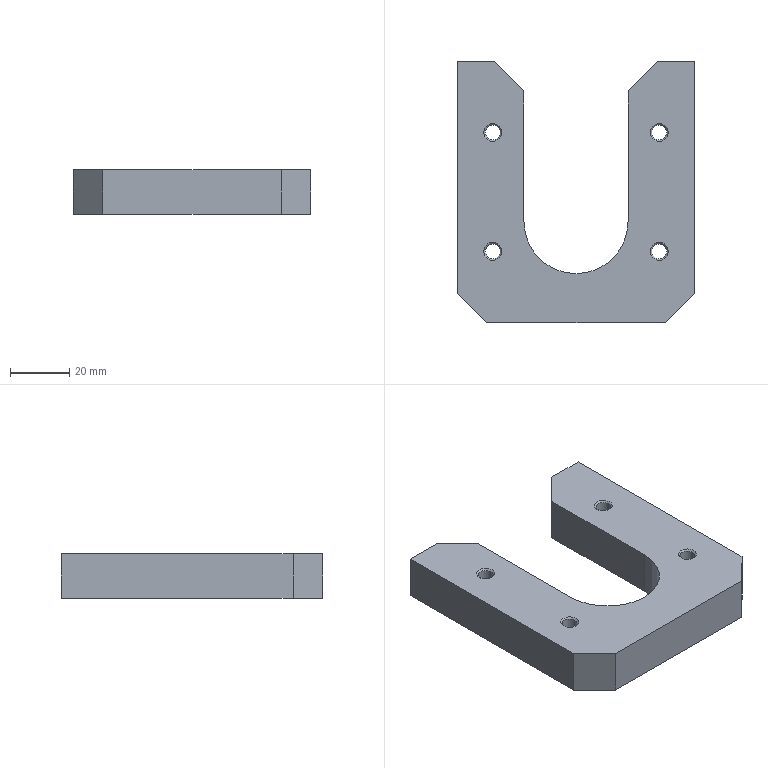Component | SolidWorks | StopBlock-2 | 1 solid | 30 faces | box 80 x 88 x 15 mm | volume 65847 mm3 | plane 13 | cylinder 9 | cone 8 | commonest cylinder face diameters 5 x8 35 x1
build123d program:
from build123d import *

# Parameters (mm, degrees)
SKETCH1_W                = 80
SKETCH1_H                = 88
BOSS_EXTRUDE1_DEPTH      = 15
CUT_EXTRUDE1_DEPTH       = 98.821
F_5_0_5_DIAMETER_HOLE1_D = 5
CHAMFER1_SIZE            = 0.525
CHAMFER2_SIZE            = 10


with BuildPart() as part:
    # Sketch1 → Boss-Extrude1 (new body)
    with BuildSketch(Plane.XY.offset(7.5)):
        with Locations((0, 44)):
            Rectangle(SKETCH1_W, SKETCH1_H)
    extrude(amount=-BOSS_EXTRUDE1_DEPTH)

    # Sketch2 → Cut-Extrude1 (cut, through all)
    with BuildSketch(Plane(origin=(0, 0, -7.5), x_dir=(-1, 0, 0), z_dir=(0, 0, -1))):
        with BuildLine():
            Line((-27.5, 88), (-17.5, 78))
            Line((-17.5, 78), (-17.5, 34))
            ThreePointArc((-17.5, 34), (0, 16.5), (17.5, 34))
            Line((17.5, 34), (17.5, 78))
            Line((17.5, 78), (27.5, 88))
            Line((27.5, 88), (-27.5, 88))
        make_face()
    extrude(amount=-CUT_EXTRUDE1_DEPTH, mode=Mode.SUBTRACT)

    # 5.0 _5_ Diameter Hole1 (through all)
    with Locations(Plane.XY.offset(7.5)):
        with Locations((-28, 24), (28, 24), (28, 64), (-28, 64)):
            Hole(F_5_0_5_DIAMETER_HOLE1_D / 2)

    # Chamfer1
    chamfer1_edges = [part.edges().sort_by_distance(p)[0] for p in [
        (-25.5, 64, 7.5),
        (30.5, 64, 7.5),
        (30.5, 24, 7.5),
        (-25.5, 24, 7.5),
    ]]
    chamfer(chamfer1_edges, length=CHAMFER1_SIZE)

    # Chamfer2
    chamfer2_edges = [part.edges().sort_by_distance(p)[0] for p in [
        (40, 0, 0),
        (-40, 0, 0),
    ]]
    chamfer(chamfer2_edges, length=CHAMFER2_SIZE)


solid = part.part

# Placed as in the assembly
solid = solid.moved(Location((-345, -263, -255), (0, 0, 0)))
STEP:
#1=CARTESIAN_POINT('',(-12.579,-7.835,-9.765));
#2=VERTEX_POINT('',#1);
#3=CARTESIAN_POINT('',(-12.382,-7.835,-9.765));
#4=VERTEX_POINT('',#3);
#5=CARTESIAN_POINT('',(-12.48,-7.835,-9.765));
#6=DIRECTION('',(0.,0.,1.));
#7=DIRECTION('',(1.,0.,0.));
#8=AXIS2_PLACEMENT_3D('',#5,#6,#7);
#9=CIRCLE('',#8,0.09843);
#10=EDGE_CURVE('',#2,#4,#9,.T.);
#11=ORIENTED_EDGE('',*,*,#10,.F.);
#12=CARTESIAN_POINT('',(-12.599,-7.835,-9.744));
#13=VERTEX_POINT('',#12);
#14=CARTESIAN_POINT('',(-12.579,-7.835,-9.765));
#15=DIRECTION('',(-0.7071,0.,0.7071));
#16=VECTOR('',#15,39.37);
#17=LINE('',#14,#16);
#18=EDGE_CURVE('',#2,#13,#17,.T.);
#19=ORIENTED_EDGE('',*,*,#18,.T.);
#20=CARTESIAN_POINT('',(-12.361,-7.835,-9.744));
#21=VERTEX_POINT('',#20);
#22=CARTESIAN_POINT('',(-12.48,-7.835,-9.744));
#23=DIRECTION('',(0.,0.,-1.));
#24=DIRECTION('',(1.,0.,0.));
#25=AXIS2_PLACEMENT_3D('',#22,#23,#24);
#26=CIRCLE('',#25,0.1191);
#27=EDGE_CURVE('',#21,#13,#26,.T.);
#28=ORIENTED_EDGE('',*,*,#27,.F.);
#29=CARTESIAN_POINT('',(-12.382,-7.835,-9.765));
#30=DIRECTION('',(0.7071,0.,0.7071));
#31=VECTOR('',#30,39.37);
#32=LINE('',#29,#31);
#33=EDGE_CURVE('',#4,#21,#32,.T.);
#34=ORIENTED_EDGE('',*,*,#33,.F.);
#35=EDGE_LOOP('',(#11,#19,#28,#34));
#36=FACE_OUTER_BOUND('',#35,.T.);
#37=CARTESIAN_POINT('',(-12.48,-7.835,-9.765));
#38=DIRECTION('',(0.,0.,1.));
#39=DIRECTION('',(1.,0.,0.));
#40=AXIS2_PLACEMENT_3D('',#37,#38,#39);
#41=CONICAL_SURFACE('',#40,0.09843,0.7854);
#42=ADVANCED_FACE('',(#36),#41,.F.);
#43=CARTESIAN_POINT('',(-14.783,-9.409,-9.765));
#44=VERTEX_POINT('',#43);
#45=CARTESIAN_POINT('',(-14.587,-9.409,-9.765));
#46=VERTEX_POINT('',#45);
#47=CARTESIAN_POINT('',(-14.685,-9.409,-9.765));
#48=DIRECTION('',(0.,0.,1.));
#49=DIRECTION('',(1.,0.,0.));
#50=AXIS2_PLACEMENT_3D('',#47,#48,#49);
#51=CIRCLE('',#50,0.09843);
#52=EDGE_CURVE('',#44,#46,#51,.T.);
#53=ORIENTED_EDGE('',*,*,#52,.F.);
#54=CARTESIAN_POINT('',(-14.804,-9.409,-9.744));
#55=VERTEX_POINT('',#54);
#56=CARTESIAN_POINT('',(-14.783,-9.409,-9.765));
#57=DIRECTION('',(-0.7071,0.,0.7071));
#58=VECTOR('',#57,39.37);
#59=LINE('',#56,#58);
#60=EDGE_CURVE('',#44,#55,#59,.T.);
#61=ORIENTED_EDGE('',*,*,#60,.T.);
#62=CARTESIAN_POINT('',(-14.566,-9.409,-9.744));
#63=VERTEX_POINT('',#62);
#64=CARTESIAN_POINT('',(-14.685,-9.409,-9.744));
#65=DIRECTION('',(0.,0.,-1.));
#66=DIRECTION('',(1.,0.,0.));
#67=AXIS2_PLACEMENT_3D('',#64,#65,#66);
#68=CIRCLE('',#67,0.1191);
#69=EDGE_CURVE('',#63,#55,#68,.T.);
#70=ORIENTED_EDGE('',*,*,#69,.F.);
#71=CARTESIAN_POINT('',(-14.587,-9.409,-9.765));
#72=DIRECTION('',(0.7071,0.,0.7071));
#73=VECTOR('',#72,39.37);
#74=LINE('',#71,#73);
#75=EDGE_CURVE('',#46,#63,#74,.T.);
#76=ORIENTED_EDGE('',*,*,#75,.F.);
#77=EDGE_LOOP('',(#53,#61,#70,#76));
#78=FACE_OUTER_BOUND('',#77,.T.);
#79=CARTESIAN_POINT('',(-14.685,-9.409,-9.765));
#80=DIRECTION('',(0.,0.,1.));
#81=DIRECTION('',(1.,0.,0.));
#82=AXIS2_PLACEMENT_3D('',#79,#80,#81);
#83=CONICAL_SURFACE('',#82,0.09843,0.7854);
#84=ADVANCED_FACE('',(#78),#83,.F.);
#85=CARTESIAN_POINT('',(-12.579,-9.409,-9.765));
#86=VERTEX_POINT('',#85);
#87=CARTESIAN_POINT('',(-12.382,-9.409,-9.765));
#88=VERTEX_POINT('',#87);
#89=CARTESIAN_POINT('',(-12.48,-9.409,-9.765));
#90=DIRECTION('',(0.,0.,1.));
#91=DIRECTION('',(1.,0.,0.));
#92=AXIS2_PLACEMENT_3D('',#89,#90,#91);
#93=CIRCLE('',#92,0.09843);
#94=EDGE_CURVE('',#86,#88,#93,.T.);
#95=ORIENTED_EDGE('',*,*,#94,.F.);
#96=CARTESIAN_POINT('',(-12.599,-9.409,-9.744));
#97=VERTEX_POINT('',#96);
#98=CARTESIAN_POINT('',(-12.579,-9.409,-9.765));
#99=DIRECTION('',(-0.7071,0.,0.7071));
#100=VECTOR('',#99,39.37);
#101=LINE('',#98,#100);
#102=EDGE_CURVE('',#86,#97,#101,.T.);
#103=ORIENTED_EDGE('',*,*,#102,.T.);
#104=CARTESIAN_POINT('',(-12.361,-9.409,-9.744));
#105=VERTEX_POINT('',#104);
#106=CARTESIAN_POINT('',(-12.48,-9.409,-9.744));
#107=DIRECTION('',(0.,0.,-1.));
#108=DIRECTION('',(1.,0.,0.));
#109=AXIS2_PLACEMENT_3D('',#106,#107,#108);
#110=CIRCLE('',#109,0.1191);
#111=EDGE_CURVE('',#105,#97,#110,.T.);
#112=ORIENTED_EDGE('',*,*,#111,.F.);
#113=CARTESIAN_POINT('',(-12.382,-9.409,-9.765));
#114=DIRECTION('',(0.7071,0.,0.7071));
#115=VECTOR('',#114,39.37);
#116=LINE('',#113,#115);
#117=EDGE_CURVE('',#88,#105,#116,.T.);
#118=ORIENTED_EDGE('',*,*,#117,.F.);
#119=EDGE_LOOP('',(#95,#103,#112,#118));
#120=FACE_OUTER_BOUND('',#119,.T.);
#121=CARTESIAN_POINT('',(-12.48,-9.409,-9.765));
#122=DIRECTION('',(0.,0.,1.));
#123=DIRECTION('',(1.,0.,0.));
#124=AXIS2_PLACEMENT_3D('',#121,#122,#123);
#125=CONICAL_SURFACE('',#124,0.09843,0.7854);
#126=ADVANCED_FACE('',(#120),#125,.F.);
#127=CARTESIAN_POINT('',(-14.783,-7.835,-9.765));
#128=VERTEX_POINT('',#127);
#129=CARTESIAN_POINT('',(-14.587,-7.835,-9.765));
#130=VERTEX_POINT('',#129);
#131=CARTESIAN_POINT('',(-14.685,-7.835,-9.765));
#132=DIRECTION('',(0.,0.,1.));
#133=DIRECTION('',(1.,0.,0.));
#134=AXIS2_PLACEMENT_3D('',#131,#132,#133);
#135=CIRCLE('',#134,0.09843);
#136=EDGE_CURVE('',#128,#130,#135,.T.);
#137=ORIENTED_EDGE('',*,*,#136,.F.);
#138=CARTESIAN_POINT('',(-14.804,-7.835,-9.744));
#139=VERTEX_POINT('',#138);
#140=CARTESIAN_POINT('',(-14.783,-7.835,-9.765));
#141=DIRECTION('',(-0.7071,0.,0.7071));
#142=VECTOR('',#141,39.37);
#143=LINE('',#140,#142);
#144=EDGE_CURVE('',#128,#139,#143,.T.);
#145=ORIENTED_EDGE('',*,*,#144,.T.);
#146=CARTESIAN_POINT('',(-14.566,-7.835,-9.744));
#147=VERTEX_POINT('',#146);
#148=CARTESIAN_POINT('',(-14.685,-7.835,-9.744));
#149=DIRECTION('',(0.,0.,-1.));
#150=DIRECTION('',(1.,0.,0.));
#151=AXIS2_PLACEMENT_3D('',#148,#149,#150);
#152=CIRCLE('',#151,0.1191);
#153=EDGE_CURVE('',#147,#139,#152,.T.);
#154=ORIENTED_EDGE('',*,*,#153,.F.);
#155=CARTESIAN_POINT('',(-14.587,-7.835,-9.765));
#156=DIRECTION('',(0.7071,0.,0.7071));
#157=VECTOR('',#156,39.37);
#158=LINE('',#155,#157);
#159=EDGE_CURVE('',#130,#147,#158,.T.);
#160=ORIENTED_EDGE('',*,*,#159,.F.);
#161=EDGE_LOOP('',(#137,#145,#154,#160));
#162=FACE_OUTER_BOUND('',#161,.T.);
#163=CARTESIAN_POINT('',(-14.685,-7.835,-9.765));
#164=DIRECTION('',(0.,0.,1.));
#165=DIRECTION('',(1.,0.,0.));
#166=AXIS2_PLACEMENT_3D('',#163,#164,#165);
#167=CONICAL_SURFACE('',#166,0.09843,0.7854);
#168=ADVANCED_FACE('',(#162),#167,.F.);
#169=CARTESIAN_POINT('',(-14.783,-9.409,-10.335));
#170=VERTEX_POINT('',#169);
#171=CARTESIAN_POINT('',(-14.587,-9.409,-10.335));
#172=VERTEX_POINT('',#171);
#173=CARTESIAN_POINT('',(-14.685,-9.409,-10.335));
#174=DIRECTION('',(0.,0.,1.));
#175=DIRECTION('',(1.,0.,0.));
#176=AXIS2_PLACEMENT_3D('',#173,#174,#175);
#177=CIRCLE('',#176,0.09843);
#178=EDGE_CURVE('',#170,#172,#177,.T.);
#179=ORIENTED_EDGE('',*,*,#178,.F.);
#180=CARTESIAN_POINT('',(-14.783,-9.409,-9.744));
#181=DIRECTION('',(0.,0.,1.));
#182=VECTOR('',#181,39.37);
#183=LINE('',#180,#182);
#184=EDGE_CURVE('',#170,#44,#183,.T.);
#185=ORIENTED_EDGE('',*,*,#184,.T.);
#186=ORIENTED_EDGE('',*,*,#52,.T.);
#187=CARTESIAN_POINT('',(-14.587,-9.409,-9.744));
#188=DIRECTION('',(0.,0.,1.));
#189=VECTOR('',#188,39.37);
#190=LINE('',#187,#189);
#191=EDGE_CURVE('',#172,#46,#190,.T.);
#192=ORIENTED_EDGE('',*,*,#191,.F.);
#193=EDGE_LOOP('',(#179,#185,#186,#192));
#194=FACE_OUTER_BOUND('',#193,.T.);
#195=CARTESIAN_POINT('',(-14.685,-9.409,-9.744));
#196=DIRECTION('',(0.,0.,1.));
#197=DIRECTION('',(1.,0.,0.));
#198=AXIS2_PLACEMENT_3D('',#195,#196,#197);
#199=CYLINDRICAL_SURFACE('',#198,0.09843);
#200=ADVANCED_FACE('',(#194),#199,.F.);
#201=CARTESIAN_POINT('',(-12.579,-9.409,-10.335));
#202=VERTEX_POINT('',#201);
#203=CARTESIAN_POINT('',(-12.382,-9.409,-10.335));
#204=VERTEX_POINT('',#203);
#205=CARTESIAN_POINT('',(-12.48,-9.409,-10.335));
#206=DIRECTION('',(0.,0.,1.));
#207=DIRECTION('',(1.,0.,0.));
#208=AXIS2_PLACEMENT_3D('',#205,#206,#207);
#209=CIRCLE('',#208,0.09843);
#210=EDGE_CURVE('',#202,#204,#209,.T.);
#211=ORIENTED_EDGE('',*,*,#210,.F.);
#212=CARTESIAN_POINT('',(-12.579,-9.409,-9.744));
#213=DIRECTION('',(0.,0.,1.));
#214=VECTOR('',#213,39.37);
#215=LINE('',#212,#214);
#216=EDGE_CURVE('',#202,#86,#215,.T.);
#217=ORIENTED_EDGE('',*,*,#216,.T.);
#218=ORIENTED_EDGE('',*,*,#94,.T.);
#219=CARTESIAN_POINT('',(-12.382,-9.409,-9.744));
#220=DIRECTION('',(0.,0.,1.));
#221=VECTOR('',#220,39.37);
#222=LINE('',#219,#221);
#223=EDGE_CURVE('',#204,#88,#222,.T.);
#224=ORIENTED_EDGE('',*,*,#223,.F.);
#225=EDGE_LOOP('',(#211,#217,#218,#224));
#226=FACE_OUTER_BOUND('',#225,.T.);
#227=CARTESIAN_POINT('',(-12.48,-9.409,-9.744));
#228=DIRECTION('',(0.,0.,1.));
#229=DIRECTION('',(1.,0.,0.));
#230=AXIS2_PLACEMENT_3D('',#227,#228,#229);
#231=CYLINDRICAL_SURFACE('',#230,0.09843);
#232=ADVANCED_FACE('',(#226),#231,.F.);
#233=CARTESIAN_POINT('',(-12.579,-7.835,-10.335));
#234=VERTEX_POINT('',#233);
#235=CARTESIAN_POINT('',(-12.382,-7.835,-10.335));
#236=VERTEX_POINT('',#235);
#237=CARTESIAN_POINT('',(-12.48,-7.835,-10.335));
#238=DIRECTION('',(0.,0.,1.));
#239=DIRECTION('',(1.,0.,0.));
#240=AXIS2_PLACEMENT_3D('',#237,#238,#239);
#241=CIRCLE('',#240,0.09843);
#242=EDGE_CURVE('',#234,#236,#241,.T.);
#243=ORIENTED_EDGE('',*,*,#242,.F.);
#244=CARTESIAN_POINT('',(-12.579,-7.835,-9.744));
#245=DIRECTION('',(0.,0.,1.));
#246=VECTOR('',#245,39.37);
#247=LINE('',#244,#246);
#248=EDGE_CURVE('',#234,#2,#247,.T.);
#249=ORIENTED_EDGE('',*,*,#248,.T.);
#250=ORIENTED_EDGE('',*,*,#10,.T.);
#251=CARTESIAN_POINT('',(-12.382,-7.835,-9.744));
#252=DIRECTION('',(0.,0.,1.));
#253=VECTOR('',#252,39.37);
#254=LINE('',#251,#253);
#255=EDGE_CURVE('',#236,#4,#254,.T.);
#256=ORIENTED_EDGE('',*,*,#255,.F.);
#257=EDGE_LOOP('',(#243,#249,#250,#256));
#258=FACE_OUTER_BOUND('',#257,.T.);
#259=CARTESIAN_POINT('',(-12.48,-7.835,-9.744));
#260=DIRECTION('',(0.,0.,1.));
#261=DIRECTION('',(1.,0.,0.));
#262=AXIS2_PLACEMENT_3D('',#259,#260,#261);
#263=CYLINDRICAL_SURFACE('',#262,0.09843);
#264=ADVANCED_FACE('',(#258),#263,.F.);
#265=CARTESIAN_POINT('',(-14.783,-7.835,-10.335));
#266=VERTEX_POINT('',#265);
#267=CARTESIAN_POINT('',(-14.587,-7.835,-10.335));
#268=VERTEX_POINT('',#267);
#269=CARTESIAN_POINT('',(-14.685,-7.835,-10.335));
#270=DIRECTION('',(0.,0.,1.));
#271=DIRECTION('',(1.,0.,0.));
#272=AXIS2_PLACEMENT_3D('',#269,#270,#271);
#273=CIRCLE('',#272,0.09843);
#274=EDGE_CURVE('',#266,#268,#273,.T.);
#275=ORIENTED_EDGE('',*,*,#274,.F.);
#276=CARTESIAN_POINT('',(-14.783,-7.835,-9.744));
#277=DIRECTION('',(0.,0.,1.));
#278=VECTOR('',#277,39.37);
#279=LINE('',#276,#278);
#280=EDGE_CURVE('',#266,#128,#279,.T.);
#281=ORIENTED_EDGE('',*,*,#280,.T.);
#282=ORIENTED_EDGE('',*,*,#136,.T.);
#283=CARTESIAN_POINT('',(-14.587,-7.835,-9.744));
#284=DIRECTION('',(0.,0.,1.));
#285=VECTOR('',#284,39.37);
#286=LINE('',#283,#285);
#287=EDGE_CURVE('',#268,#130,#286,.T.);
#288=ORIENTED_EDGE('',*,*,#287,.F.);
#289=EDGE_LOOP('',(#275,#281,#282,#288));
#290=FACE_OUTER_BOUND('',#289,.T.);
#291=CARTESIAN_POINT('',(-14.685,-7.835,-9.744));
#292=DIRECTION('',(0.,0.,1.));
#293=DIRECTION('',(1.,0.,0.));
#294=AXIS2_PLACEMENT_3D('',#291,#292,#293);
#295=CYLINDRICAL_SURFACE('',#294,0.09843);
#296=ADVANCED_FACE('',(#290),#295,.F.);
#297=CARTESIAN_POINT('',(-14.665,-6.89,-9.744));
#298=VERTEX_POINT('',#297);
#299=CARTESIAN_POINT('',(-14.665,-6.89,-10.335));
#300=VERTEX_POINT('',#299);
#301=CARTESIAN_POINT('',(-14.665,-6.89,-9.744));
#302=DIRECTION('',(0.,0.,-1.));
#303=VECTOR('',#302,39.37);
#304=LINE('',#301,#303);
#305=EDGE_CURVE('',#298,#300,#304,.T.);
#306=ORIENTED_EDGE('',*,*,#305,.T.);
#307=CARTESIAN_POINT('',(-15.157,-6.89,-10.335));
#308=VERTEX_POINT('',#307);
#309=CARTESIAN_POINT('',(-12.008,-6.89,-10.335));
#310=DIRECTION('',(-1.,0.,0.));
#311=VECTOR('',#310,39.37);
#312=LINE('',#309,#311);
#313=EDGE_CURVE('',#300,#308,#312,.T.);
#314=ORIENTED_EDGE('',*,*,#313,.T.);
#315=CARTESIAN_POINT('',(-15.157,-6.89,-9.744));
#316=VERTEX_POINT('',#315);
#317=CARTESIAN_POINT('',(-15.157,-6.89,-10.335));
#318=DIRECTION('',(0.,0.,1.));
#319=VECTOR('',#318,39.37);
#320=LINE('',#317,#319);
#321=EDGE_CURVE('',#308,#316,#320,.T.);
#322=ORIENTED_EDGE('',*,*,#321,.T.);
#323=CARTESIAN_POINT('',(-12.008,-6.89,-9.744));
#324=DIRECTION('',(-1.,0.,0.));
#325=VECTOR('',#324,39.37);
#326=LINE('',#323,#325);
#327=EDGE_CURVE('',#298,#316,#326,.T.);
#328=ORIENTED_EDGE('',*,*,#327,.F.);
#329=EDGE_LOOP('',(#306,#314,#322,#328));
#330=FACE_OUTER_BOUND('',#329,.T.);
#331=CARTESIAN_POINT('',(-12.008,-6.89,-10.335));
#332=DIRECTION('',(0.,1.,0.));
#333=DIRECTION('',(0.,0.,1.));
#334=AXIS2_PLACEMENT_3D('',#331,#332,#333);
#335=PLANE('',#334);
#336=ADVANCED_FACE('',(#330),#335,.T.);
#337=CARTESIAN_POINT('',(-12.008,-9.961,-9.744));
#338=VERTEX_POINT('',#337);
#339=CARTESIAN_POINT('',(-12.008,-6.89,-9.744));
#340=VERTEX_POINT('',#339);
#341=CARTESIAN_POINT('',(-12.008,-10.354,-9.744));
#342=DIRECTION('',(-0.,1.,0.));
#343=VECTOR('',#342,39.37);
#344=LINE('',#341,#343);
#345=EDGE_CURVE('',#338,#340,#344,.T.);
#346=ORIENTED_EDGE('',*,*,#345,.F.);
#347=CARTESIAN_POINT('',(-12.008,-9.961,-10.335));
#348=VERTEX_POINT('',#347);
#349=CARTESIAN_POINT('',(-12.008,-9.961,-10.335));
#350=DIRECTION('',(0.,0.,-1.));
#351=VECTOR('',#350,39.37);
#352=LINE('',#349,#351);
#353=EDGE_CURVE('',#338,#348,#352,.T.);
#354=ORIENTED_EDGE('',*,*,#353,.T.);
#355=CARTESIAN_POINT('',(-12.008,-6.89,-10.335));
#356=VERTEX_POINT('',#355);
#357=CARTESIAN_POINT('',(-12.008,-10.354,-10.335));
#358=DIRECTION('',(-0.,1.,0.));
#359=VECTOR('',#358,39.37);
#360=LINE('',#357,#359);
#361=EDGE_CURVE('',#348,#356,#360,.T.);
#362=ORIENTED_EDGE('',*,*,#361,.T.);
#363=CARTESIAN_POINT('',(-12.008,-6.89,-10.335));
#364=DIRECTION('',(0.,0.,1.));
#365=VECTOR('',#364,39.37);
#366=LINE('',#363,#365);
#367=EDGE_CURVE('',#356,#340,#366,.T.);
#368=ORIENTED_EDGE('',*,*,#367,.T.);
#369=EDGE_LOOP('',(#346,#354,#362,#368));
#370=FACE_OUTER_BOUND('',#369,.T.);
#371=CARTESIAN_POINT('',(-12.008,-10.354,-10.335));
#372=DIRECTION('',(1.,0.,0.));
#373=DIRECTION('',(-0.,1.,0.));
#374=AXIS2_PLACEMENT_3D('',#371,#372,#373);
#375=PLANE('',#374);
#376=ADVANCED_FACE('',(#370),#375,.T.);
#377=CARTESIAN_POINT('',(-14.764,-10.354,-10.335));
#378=VERTEX_POINT('',#377);
#379=CARTESIAN_POINT('',(-12.402,-10.354,-10.335));
#380=VERTEX_POINT('',#379);
#381=CARTESIAN_POINT('',(-15.157,-10.354,-10.335));
#382=DIRECTION('',(1.,0.,0.));
#383=VECTOR('',#382,39.37);
#384=LINE('',#381,#383);
#385=EDGE_CURVE('',#378,#380,#384,.T.);
#386=ORIENTED_EDGE('',*,*,#385,.T.);
#387=CARTESIAN_POINT('',(-12.402,-10.354,-9.744));
#388=VERTEX_POINT('',#387);
#389=CARTESIAN_POINT('',(-12.402,-10.354,-10.335));
#390=DIRECTION('',(0.,0.,1.));
#391=VECTOR('',#390,39.37);
#392=LINE('',#389,#391);
#393=EDGE_CURVE('',#380,#388,#392,.T.);
#394=ORIENTED_EDGE('',*,*,#393,.T.);
#395=CARTESIAN_POINT('',(-14.764,-10.354,-9.744));
#396=VERTEX_POINT('',#395);
#397=CARTESIAN_POINT('',(-15.157,-10.354,-9.744));
#398=DIRECTION('',(1.,0.,0.));
#399=VECTOR('',#398,39.37);
#400=LINE('',#397,#399);
#401=EDGE_CURVE('',#396,#388,#400,.T.);
#402=ORIENTED_EDGE('',*,*,#401,.F.);
#403=CARTESIAN_POINT('',(-14.764,-10.354,-10.335));
#404=DIRECTION('',(0.,0.,-1.));
#405=VECTOR('',#404,39.37);
#406=LINE('',#403,#405);
#407=EDGE_CURVE('',#396,#378,#406,.T.);
#408=ORIENTED_EDGE('',*,*,#407,.T.);
#409=EDGE_LOOP('',(#386,#394,#402,#408));
#410=FACE_OUTER_BOUND('',#409,.T.);
#411=CARTESIAN_POINT('',(-15.157,-10.354,-10.335));
#412=DIRECTION('',(0.,-1.,0.));
#413=DIRECTION('',(0.,0.,-1.));
#414=AXIS2_PLACEMENT_3D('',#411,#412,#413);
#415=PLANE('',#414);
#416=ADVANCED_FACE('',(#410),#415,.T.);
#417=CARTESIAN_POINT('',(-15.157,-9.961,-10.335));
#418=VERTEX_POINT('',#417);
#419=CARTESIAN_POINT('',(-15.157,-6.89,-10.335));
#420=DIRECTION('',(0.,-1.,0.));
#421=VECTOR('',#420,39.37);
#422=LINE('',#419,#421);
#423=EDGE_CURVE('',#308,#418,#422,.T.);
#424=ORIENTED_EDGE('',*,*,#423,.T.);
#425=CARTESIAN_POINT('',(-15.157,-9.961,-9.744));
#426=VERTEX_POINT('',#425);
#427=CARTESIAN_POINT('',(-15.157,-9.961,-10.335));
#428=DIRECTION('',(0.,0.,1.));
#429=VECTOR('',#428,39.37);
#430=LINE('',#427,#429);
#431=EDGE_CURVE('',#418,#426,#430,.T.);
#432=ORIENTED_EDGE('',*,*,#431,.T.);
#433=CARTESIAN_POINT('',(-15.157,-6.89,-9.744));
#434=DIRECTION('',(0.,-1.,0.));
#435=VECTOR('',#434,39.37);
#436=LINE('',#433,#435);
#437=EDGE_CURVE('',#316,#426,#436,.T.);
#438=ORIENTED_EDGE('',*,*,#437,.F.);
#439=ORIENTED_EDGE('',*,*,#321,.F.);
#440=EDGE_LOOP('',(#424,#432,#438,#439));
#441=FACE_OUTER_BOUND('',#440,.T.);
#442=CARTESIAN_POINT('',(-15.157,-6.89,-10.335));
#443=DIRECTION('',(-1.,0.,0.));
#444=DIRECTION('',(0.,0.,1.));
#445=AXIS2_PLACEMENT_3D('',#442,#443,#444);
#446=PLANE('',#445);
#447=ADVANCED_FACE('',(#441),#446,.T.);
#448=CARTESIAN_POINT('',(-12.5,-6.89,-9.744));
#449=VERTEX_POINT('',#448);
#450=CARTESIAN_POINT('',(-12.5,-6.89,-10.335));
#451=VERTEX_POINT('',#450);
#452=CARTESIAN_POINT('',(-12.5,-6.89,-9.744));
#453=DIRECTION('',(0.,0.,-1.));
#454=VECTOR('',#453,39.37);
#455=LINE('',#452,#454);
#456=EDGE_CURVE('',#449,#451,#455,.T.);
#457=ORIENTED_EDGE('',*,*,#456,.F.);
#458=CARTESIAN_POINT('',(-12.008,-6.89,-9.744));
#459=DIRECTION('',(-1.,0.,0.));
#460=VECTOR('',#459,39.37);
#461=LINE('',#458,#460);
#462=EDGE_CURVE('',#340,#449,#461,.T.);
#463=ORIENTED_EDGE('',*,*,#462,.F.);
#464=ORIENTED_EDGE('',*,*,#367,.F.);
#465=CARTESIAN_POINT('',(-12.008,-6.89,-10.335));
#466=DIRECTION('',(-1.,0.,0.));
#467=VECTOR('',#466,39.37);
#468=LINE('',#465,#467);
#469=EDGE_CURVE('',#356,#451,#468,.T.);
#470=ORIENTED_EDGE('',*,*,#469,.T.);
#471=EDGE_LOOP('',(#457,#463,#464,#470));
#472=FACE_OUTER_BOUND('',#471,.T.);
#473=CARTESIAN_POINT('',(-12.008,-6.89,-10.335));
#474=DIRECTION('',(0.,1.,0.));
#475=DIRECTION('',(0.,0.,1.));
#476=AXIS2_PLACEMENT_3D('',#473,#474,#475);
#477=PLANE('',#476);
#478=ADVANCED_FACE('',(#472),#477,.T.);
#479=CARTESIAN_POINT('',(-14.685,-9.409,-10.335));
#480=DIRECTION('',(0.,0.,1.));
#481=DIRECTION('',(1.,0.,0.));
#482=AXIS2_PLACEMENT_3D('',#479,#480,#481);
#483=CIRCLE('',#482,0.09843);
#484=EDGE_CURVE('',#172,#170,#483,.T.);
#485=ORIENTED_EDGE('',*,*,#484,.T.);
#486=ORIENTED_EDGE('',*,*,#178,.T.);
#487=EDGE_LOOP('',(#485,#486));
#488=FACE_BOUND('',#487,.T.);
#489=CARTESIAN_POINT('',(-12.48,-9.409,-10.335));
#490=DIRECTION('',(0.,0.,1.));
#491=DIRECTION('',(1.,0.,0.));
#492=AXIS2_PLACEMENT_3D('',#489,#490,#491);
#493=CIRCLE('',#492,0.09843);
#494=EDGE_CURVE('',#204,#202,#493,.T.);
#495=ORIENTED_EDGE('',*,*,#494,.T.);
#496=ORIENTED_EDGE('',*,*,#210,.T.);
#497=EDGE_LOOP('',(#495,#496));
#498=FACE_BOUND('',#497,.T.);
#499=CARTESIAN_POINT('',(-12.48,-7.835,-10.335));
#500=DIRECTION('',(0.,0.,1.));
#501=DIRECTION('',(1.,0.,0.));
#502=AXIS2_PLACEMENT_3D('',#499,#500,#501);
#503=CIRCLE('',#502,0.09843);
#504=EDGE_CURVE('',#236,#234,#503,.T.);
#505=ORIENTED_EDGE('',*,*,#504,.T.);
#506=ORIENTED_EDGE('',*,*,#242,.T.);
#507=EDGE_LOOP('',(#505,#506));
#508=FACE_BOUND('',#507,.T.);
#509=CARTESIAN_POINT('',(-14.685,-7.835,-10.335));
#510=DIRECTION('',(0.,0.,1.));
#511=DIRECTION('',(1.,0.,0.));
#512=AXIS2_PLACEMENT_3D('',#509,#510,#511);
#513=CIRCLE('',#512,0.09843);
#514=EDGE_CURVE('',#268,#266,#513,.T.);
#515=ORIENTED_EDGE('',*,*,#514,.T.);
#516=ORIENTED_EDGE('',*,*,#274,.T.);
#517=EDGE_LOOP('',(#515,#516));
#518=FACE_BOUND('',#517,.T.);
#519=ORIENTED_EDGE('',*,*,#361,.F.);
#520=CARTESIAN_POINT('',(-12.402,-10.354,-10.335));
#521=DIRECTION('',(-0.7071,-0.7071,0.));
#522=VECTOR('',#521,39.37);
#523=LINE('',#520,#522);
#524=EDGE_CURVE('',#348,#380,#523,.T.);
#525=ORIENTED_EDGE('',*,*,#524,.T.);
#526=ORIENTED_EDGE('',*,*,#385,.F.);
#527=CARTESIAN_POINT('',(-15.157,-9.961,-10.335));
#528=DIRECTION('',(-0.7071,0.7071,0.));
#529=VECTOR('',#528,39.37);
#530=LINE('',#527,#529);
#531=EDGE_CURVE('',#378,#418,#530,.T.);
#532=ORIENTED_EDGE('',*,*,#531,.T.);
#533=ORIENTED_EDGE('',*,*,#423,.F.);
#534=ORIENTED_EDGE('',*,*,#313,.F.);
#535=CARTESIAN_POINT('',(-14.272,-7.283,-10.335));
#536=VERTEX_POINT('',#535);
#537=CARTESIAN_POINT('',(-14.272,-7.283,-10.335));
#538=DIRECTION('',(-0.7071,0.7071,0.));
#539=VECTOR('',#538,39.37);
#540=LINE('',#537,#539);
#541=EDGE_CURVE('',#536,#300,#540,.T.);
#542=ORIENTED_EDGE('',*,*,#541,.F.);
#543=CARTESIAN_POINT('',(-14.272,-9.016,-10.335));
#544=VERTEX_POINT('',#543);
#545=CARTESIAN_POINT('',(-14.272,-9.016,-10.335));
#546=DIRECTION('',(0.,1.,0.));
#547=VECTOR('',#546,39.37);
#548=LINE('',#545,#547);
#549=EDGE_CURVE('',#544,#536,#548,.T.);
#550=ORIENTED_EDGE('',*,*,#549,.F.);
#551=CARTESIAN_POINT('',(-12.894,-9.016,-10.335));
#552=VERTEX_POINT('',#551);
#553=CARTESIAN_POINT('',(-13.583,-9.016,-10.335));
#554=DIRECTION('',(0.,0.,-1.));
#555=DIRECTION('',(-1.,0.,0.));
#556=AXIS2_PLACEMENT_3D('',#553,#554,#555);
#557=CIRCLE('',#556,0.689);
#558=EDGE_CURVE('',#552,#544,#557,.T.);
#559=ORIENTED_EDGE('',*,*,#558,.F.);
#560=CARTESIAN_POINT('',(-12.894,-7.283,-10.335));
#561=VERTEX_POINT('',#560);
#562=CARTESIAN_POINT('',(-12.894,-7.283,-10.335));
#563=DIRECTION('',(0.,-1.,0.));
#564=VECTOR('',#563,39.37);
#565=LINE('',#562,#564);
#566=EDGE_CURVE('',#561,#552,#565,.T.);
#567=ORIENTED_EDGE('',*,*,#566,.F.);
#568=CARTESIAN_POINT('',(-12.5,-6.89,-10.335));
#569=DIRECTION('',(-0.7071,-0.7071,0.));
#570=VECTOR('',#569,39.37);
#571=LINE('',#568,#570);
#572=EDGE_CURVE('',#451,#561,#571,.T.);
#573=ORIENTED_EDGE('',*,*,#572,.F.);
#574=ORIENTED_EDGE('',*,*,#469,.F.);
#575=EDGE_LOOP('',(#519,#525,#526,#532,#533,#534,#542,#550,#559,#567,#573,#574));
#576=FACE_OUTER_BOUND('',#575,.T.);
#577=CARTESIAN_POINT('',(-13.583,-10.354,-10.335));
#578=DIRECTION('',(0.,0.,1.));
#579=DIRECTION('',(1.,0.,0.));
#580=AXIS2_PLACEMENT_3D('',#577,#578,#579);
#581=PLANE('',#580);
#582=ADVANCED_FACE('',(#488,#498,#508,#518,#576),#581,.F.);
#583=ORIENTED_EDGE('',*,*,#153,.T.);
#584=CARTESIAN_POINT('',(-14.685,-7.835,-9.744));
#585=DIRECTION('',(0.,0.,-1.));
#586=DIRECTION('',(1.,0.,0.));
#587=AXIS2_PLACEMENT_3D('',#584,#585,#586);
#588=CIRCLE('',#587,0.1191);
#589=EDGE_CURVE('',#139,#147,#588,.T.);
#590=ORIENTED_EDGE('',*,*,#589,.T.);
#591=EDGE_LOOP('',(#583,#590));
#592=FACE_BOUND('',#591,.T.);
#593=ORIENTED_EDGE('',*,*,#111,.T.);
#594=CARTESIAN_POINT('',(-12.48,-9.409,-9.744));
#595=DIRECTION('',(0.,0.,-1.));
#596=DIRECTION('',(1.,0.,0.));
#597=AXIS2_PLACEMENT_3D('',#594,#595,#596);
#598=CIRCLE('',#597,0.1191);
#599=EDGE_CURVE('',#97,#105,#598,.T.);
#600=ORIENTED_EDGE('',*,*,#599,.T.);
#601=EDGE_LOOP('',(#593,#600));
#602=FACE_BOUND('',#601,.T.);
#603=ORIENTED_EDGE('',*,*,#69,.T.);
#604=CARTESIAN_POINT('',(-14.685,-9.409,-9.744));
#605=DIRECTION('',(0.,0.,-1.));
#606=DIRECTION('',(1.,0.,0.));
#607=AXIS2_PLACEMENT_3D('',#604,#605,#606);
#608=CIRCLE('',#607,0.1191);
#609=EDGE_CURVE('',#55,#63,#608,.T.);
#610=ORIENTED_EDGE('',*,*,#609,.T.);
#611=EDGE_LOOP('',(#603,#610));
#612=FACE_BOUND('',#611,.T.);
#613=ORIENTED_EDGE('',*,*,#27,.T.);
#614=CARTESIAN_POINT('',(-12.48,-7.835,-9.744));
#615=DIRECTION('',(0.,0.,-1.));
#616=DIRECTION('',(1.,0.,0.));
#617=AXIS2_PLACEMENT_3D('',#614,#615,#616);
#618=CIRCLE('',#617,0.1191);
#619=EDGE_CURVE('',#13,#21,#618,.T.);
#620=ORIENTED_EDGE('',*,*,#619,.T.);
#621=EDGE_LOOP('',(#613,#620));
#622=FACE_BOUND('',#621,.T.);
#623=ORIENTED_EDGE('',*,*,#401,.T.);
#624=CARTESIAN_POINT('',(-12.992,-10.945,-9.744));
#625=DIRECTION('',(0.7071,0.7071,0.));
#626=VECTOR('',#625,39.37);
#627=LINE('',#624,#626);
#628=EDGE_CURVE('',#388,#338,#627,.T.);
#629=ORIENTED_EDGE('',*,*,#628,.T.);
#630=ORIENTED_EDGE('',*,*,#345,.T.);
#631=ORIENTED_EDGE('',*,*,#462,.T.);
#632=CARTESIAN_POINT('',(-12.894,-7.283,-9.744));
#633=VERTEX_POINT('',#632);
#634=CARTESIAN_POINT('',(-12.5,-6.89,-9.744));
#635=DIRECTION('',(-0.7071,-0.7071,0.));
#636=VECTOR('',#635,39.37);
#637=LINE('',#634,#636);
#638=EDGE_CURVE('',#449,#633,#637,.T.);
#639=ORIENTED_EDGE('',*,*,#638,.T.);
#640=CARTESIAN_POINT('',(-12.894,-9.016,-9.744));
#641=VERTEX_POINT('',#640);
#642=CARTESIAN_POINT('',(-12.894,-7.283,-9.744));
#643=DIRECTION('',(0.,-1.,0.));
#644=VECTOR('',#643,39.37);
#645=LINE('',#642,#644);
#646=EDGE_CURVE('',#633,#641,#645,.T.);
#647=ORIENTED_EDGE('',*,*,#646,.T.);
#648=CARTESIAN_POINT('',(-14.272,-9.016,-9.744));
#649=VERTEX_POINT('',#648);
#650=CARTESIAN_POINT('',(-13.583,-9.016,-9.744));
#651=DIRECTION('',(0.,0.,-1.));
#652=DIRECTION('',(-1.,0.,0.));
#653=AXIS2_PLACEMENT_3D('',#650,#651,#652);
#654=CIRCLE('',#653,0.689);
#655=EDGE_CURVE('',#641,#649,#654,.T.);
#656=ORIENTED_EDGE('',*,*,#655,.T.);
#657=CARTESIAN_POINT('',(-14.272,-7.283,-9.744));
#658=VERTEX_POINT('',#657);
#659=CARTESIAN_POINT('',(-14.272,-9.016,-9.744));
#660=DIRECTION('',(0.,1.,0.));
#661=VECTOR('',#660,39.37);
#662=LINE('',#659,#661);
#663=EDGE_CURVE('',#649,#658,#662,.T.);
#664=ORIENTED_EDGE('',*,*,#663,.T.);
#665=CARTESIAN_POINT('',(-14.272,-7.283,-9.744));
#666=DIRECTION('',(-0.7071,0.7071,0.));
#667=VECTOR('',#666,39.37);
#668=LINE('',#665,#667);
#669=EDGE_CURVE('',#658,#298,#668,.T.);
#670=ORIENTED_EDGE('',*,*,#669,.T.);
#671=ORIENTED_EDGE('',*,*,#327,.T.);
#672=ORIENTED_EDGE('',*,*,#437,.T.);
#673=CARTESIAN_POINT('',(-14.173,-10.945,-9.744));
#674=DIRECTION('',(0.7071,-0.7071,0.));
#675=VECTOR('',#674,39.37);
#676=LINE('',#673,#675);
#677=EDGE_CURVE('',#426,#396,#676,.T.);
#678=ORIENTED_EDGE('',*,*,#677,.T.);
#679=EDGE_LOOP('',(#623,#629,#630,#631,#639,#647,#656,#664,#670,#671,#672,#678));
#680=FACE_OUTER_BOUND('',#679,.T.);
#681=CARTESIAN_POINT('',(-13.583,-10.354,-9.744));
#682=DIRECTION('',(0.,0.,1.));
#683=DIRECTION('',(1.,0.,0.));
#684=AXIS2_PLACEMENT_3D('',#681,#682,#683);
#685=PLANE('',#684);
#686=ADVANCED_FACE('',(#592,#602,#612,#622,#680),#685,.T.);
#687=ORIENTED_EDGE('',*,*,#541,.T.);
#688=ORIENTED_EDGE('',*,*,#305,.F.);
#689=ORIENTED_EDGE('',*,*,#669,.F.);
#690=CARTESIAN_POINT('',(-14.272,-7.283,-9.744));
#691=DIRECTION('',(0.,0.,-1.));
#692=VECTOR('',#691,39.37);
#693=LINE('',#690,#692);
#694=EDGE_CURVE('',#658,#536,#693,.T.);
#695=ORIENTED_EDGE('',*,*,#694,.T.);
#696=EDGE_LOOP('',(#687,#688,#689,#695));
#697=FACE_OUTER_BOUND('',#696,.T.);
#698=CARTESIAN_POINT('',(-14.272,-7.283,-9.744));
#699=DIRECTION('',(-0.7071,-0.7071,0.));
#700=DIRECTION('',(0.7071,-0.7071,0.));
#701=AXIS2_PLACEMENT_3D('',#698,#699,#700);
#702=PLANE('',#701);
#703=ADVANCED_FACE('',(#697),#702,.F.);
#704=ORIENTED_EDGE('',*,*,#549,.T.);
#705=ORIENTED_EDGE('',*,*,#694,.F.);
#706=ORIENTED_EDGE('',*,*,#663,.F.);
#707=CARTESIAN_POINT('',(-14.272,-9.016,-9.744));
#708=DIRECTION('',(0.,0.,-1.));
#709=VECTOR('',#708,39.37);
#710=LINE('',#707,#709);
#711=EDGE_CURVE('',#649,#544,#710,.T.);
#712=ORIENTED_EDGE('',*,*,#711,.T.);
#713=EDGE_LOOP('',(#704,#705,#706,#712));
#714=FACE_OUTER_BOUND('',#713,.T.);
#715=CARTESIAN_POINT('',(-14.272,-9.016,-9.744));
#716=DIRECTION('',(-1.,0.,0.));
#717=DIRECTION('',(-0.,-1.,0.));
#718=AXIS2_PLACEMENT_3D('',#715,#716,#717);
#719=PLANE('',#718);
#720=ADVANCED_FACE('',(#714),#719,.F.);
#721=ORIENTED_EDGE('',*,*,#558,.T.);
#722=ORIENTED_EDGE('',*,*,#711,.F.);
#723=ORIENTED_EDGE('',*,*,#655,.F.);
#724=CARTESIAN_POINT('',(-12.894,-9.016,-9.744));
#725=DIRECTION('',(0.,0.,-1.));
#726=VECTOR('',#725,39.37);
#727=LINE('',#724,#726);
#728=EDGE_CURVE('',#641,#552,#727,.T.);
#729=ORIENTED_EDGE('',*,*,#728,.T.);
#730=EDGE_LOOP('',(#721,#722,#723,#729));
#731=FACE_OUTER_BOUND('',#730,.T.);
#732=CARTESIAN_POINT('',(-13.583,-9.016,-9.744));
#733=DIRECTION('',(0.,0.,-1.));
#734=DIRECTION('',(-1.,0.,0.));
#735=AXIS2_PLACEMENT_3D('',#732,#733,#734);
#736=CYLINDRICAL_SURFACE('',#735,0.689);
#737=ADVANCED_FACE('',(#731),#736,.F.);
#738=ORIENTED_EDGE('',*,*,#566,.T.);
#739=ORIENTED_EDGE('',*,*,#728,.F.);
#740=ORIENTED_EDGE('',*,*,#646,.F.);
#741=CARTESIAN_POINT('',(-12.894,-7.283,-9.744));
#742=DIRECTION('',(0.,0.,-1.));
#743=VECTOR('',#742,39.37);
#744=LINE('',#741,#743);
#745=EDGE_CURVE('',#633,#561,#744,.T.);
#746=ORIENTED_EDGE('',*,*,#745,.T.);
#747=EDGE_LOOP('',(#738,#739,#740,#746));
#748=FACE_OUTER_BOUND('',#747,.T.);
#749=CARTESIAN_POINT('',(-12.894,-7.283,-9.744));
#750=DIRECTION('',(1.,0.,0.));
#751=DIRECTION('',(0.,0.,-1.));
#752=AXIS2_PLACEMENT_3D('',#749,#750,#751);
#753=PLANE('',#752);
#754=ADVANCED_FACE('',(#748),#753,.F.);
#755=ORIENTED_EDGE('',*,*,#572,.T.);
#756=ORIENTED_EDGE('',*,*,#745,.F.);
#757=ORIENTED_EDGE('',*,*,#638,.F.);
#758=ORIENTED_EDGE('',*,*,#456,.T.);
#759=EDGE_LOOP('',(#755,#756,#757,#758));
#760=FACE_OUTER_BOUND('',#759,.T.);
#761=CARTESIAN_POINT('',(-12.5,-6.89,-9.744));
#762=DIRECTION('',(0.7071,-0.7071,0.));
#763=DIRECTION('',(0.7071,0.7071,0.));
#764=AXIS2_PLACEMENT_3D('',#761,#762,#763);
#765=PLANE('',#764);
#766=ADVANCED_FACE('',(#760),#765,.F.);
#767=ORIENTED_EDGE('',*,*,#280,.F.);
#768=ORIENTED_EDGE('',*,*,#514,.F.);
#769=ORIENTED_EDGE('',*,*,#287,.T.);
#770=CARTESIAN_POINT('',(-14.685,-7.835,-9.765));
#771=DIRECTION('',(0.,0.,1.));
#772=DIRECTION('',(1.,0.,0.));
#773=AXIS2_PLACEMENT_3D('',#770,#771,#772);
#774=CIRCLE('',#773,0.09843);
#775=EDGE_CURVE('',#130,#128,#774,.T.);
#776=ORIENTED_EDGE('',*,*,#775,.T.);
#777=EDGE_LOOP('',(#767,#768,#769,#776));
#778=FACE_OUTER_BOUND('',#777,.T.);
#779=CARTESIAN_POINT('',(-14.685,-7.835,-9.744));
#780=DIRECTION('',(0.,0.,1.));
#781=DIRECTION('',(1.,0.,0.));
#782=AXIS2_PLACEMENT_3D('',#779,#780,#781);
#783=CYLINDRICAL_SURFACE('',#782,0.09843);
#784=ADVANCED_FACE('',(#778),#783,.F.);
#785=ORIENTED_EDGE('',*,*,#248,.F.);
#786=ORIENTED_EDGE('',*,*,#504,.F.);
#787=ORIENTED_EDGE('',*,*,#255,.T.);
#788=CARTESIAN_POINT('',(-12.48,-7.835,-9.765));
#789=DIRECTION('',(0.,0.,1.));
#790=DIRECTION('',(1.,0.,0.));
#791=AXIS2_PLACEMENT_3D('',#788,#789,#790);
#792=CIRCLE('',#791,0.09843);
#793=EDGE_CURVE('',#4,#2,#792,.T.);
#794=ORIENTED_EDGE('',*,*,#793,.T.);
#795=EDGE_LOOP('',(#785,#786,#787,#794));
#796=FACE_OUTER_BOUND('',#795,.T.);
#797=CARTESIAN_POINT('',(-12.48,-7.835,-9.744));
#798=DIRECTION('',(0.,0.,1.));
#799=DIRECTION('',(1.,0.,0.));
#800=AXIS2_PLACEMENT_3D('',#797,#798,#799);
#801=CYLINDRICAL_SURFACE('',#800,0.09843);
#802=ADVANCED_FACE('',(#796),#801,.F.);
#803=ORIENTED_EDGE('',*,*,#216,.F.);
#804=ORIENTED_EDGE('',*,*,#494,.F.);
#805=ORIENTED_EDGE('',*,*,#223,.T.);
#806=CARTESIAN_POINT('',(-12.48,-9.409,-9.765));
#807=DIRECTION('',(0.,0.,1.));
#808=DIRECTION('',(1.,0.,0.));
#809=AXIS2_PLACEMENT_3D('',#806,#807,#808);
#810=CIRCLE('',#809,0.09843);
#811=EDGE_CURVE('',#88,#86,#810,.T.);
#812=ORIENTED_EDGE('',*,*,#811,.T.);
#813=EDGE_LOOP('',(#803,#804,#805,#812));
#814=FACE_OUTER_BOUND('',#813,.T.);
#815=CARTESIAN_POINT('',(-12.48,-9.409,-9.744));
#816=DIRECTION('',(0.,0.,1.));
#817=DIRECTION('',(1.,0.,0.));
#818=AXIS2_PLACEMENT_3D('',#815,#816,#817);
#819=CYLINDRICAL_SURFACE('',#818,0.09843);
#820=ADVANCED_FACE('',(#814),#819,.F.);
#821=ORIENTED_EDGE('',*,*,#184,.F.);
#822=ORIENTED_EDGE('',*,*,#484,.F.);
#823=ORIENTED_EDGE('',*,*,#191,.T.);
#824=CARTESIAN_POINT('',(-14.685,-9.409,-9.765));
#825=DIRECTION('',(0.,0.,1.));
#826=DIRECTION('',(1.,0.,0.));
#827=AXIS2_PLACEMENT_3D('',#824,#825,#826);
#828=CIRCLE('',#827,0.09843);
#829=EDGE_CURVE('',#46,#44,#828,.T.);
#830=ORIENTED_EDGE('',*,*,#829,.T.);
#831=EDGE_LOOP('',(#821,#822,#823,#830));
#832=FACE_OUTER_BOUND('',#831,.T.);
#833=CARTESIAN_POINT('',(-14.685,-9.409,-9.744));
#834=DIRECTION('',(0.,0.,1.));
#835=DIRECTION('',(1.,0.,0.));
#836=AXIS2_PLACEMENT_3D('',#833,#834,#835);
#837=CYLINDRICAL_SURFACE('',#836,0.09843);
#838=ADVANCED_FACE('',(#832),#837,.F.);
#839=ORIENTED_EDGE('',*,*,#144,.F.);
#840=ORIENTED_EDGE('',*,*,#775,.F.);
#841=ORIENTED_EDGE('',*,*,#159,.T.);
#842=ORIENTED_EDGE('',*,*,#589,.F.);
#843=EDGE_LOOP('',(#839,#840,#841,#842));
#844=FACE_OUTER_BOUND('',#843,.T.);
#845=CARTESIAN_POINT('',(-14.685,-7.835,-9.765));
#846=DIRECTION('',(0.,0.,1.));
#847=DIRECTION('',(1.,0.,0.));
#848=AXIS2_PLACEMENT_3D('',#845,#846,#847);
#849=CONICAL_SURFACE('',#848,0.09843,0.7854);
#850=ADVANCED_FACE('',(#844),#849,.F.);
#851=ORIENTED_EDGE('',*,*,#102,.F.);
#852=ORIENTED_EDGE('',*,*,#811,.F.);
#853=ORIENTED_EDGE('',*,*,#117,.T.);
#854=ORIENTED_EDGE('',*,*,#599,.F.);
#855=EDGE_LOOP('',(#851,#852,#853,#854));
#856=FACE_OUTER_BOUND('',#855,.T.);
#857=CARTESIAN_POINT('',(-12.48,-9.409,-9.765));
#858=DIRECTION('',(0.,0.,1.));
#859=DIRECTION('',(1.,0.,0.));
#860=AXIS2_PLACEMENT_3D('',#857,#858,#859);
#861=CONICAL_SURFACE('',#860,0.09843,0.7854);
#862=ADVANCED_FACE('',(#856),#861,.F.);
#863=ORIENTED_EDGE('',*,*,#60,.F.);
#864=ORIENTED_EDGE('',*,*,#829,.F.);
#865=ORIENTED_EDGE('',*,*,#75,.T.);
#866=ORIENTED_EDGE('',*,*,#609,.F.);
#867=EDGE_LOOP('',(#863,#864,#865,#866));
#868=FACE_OUTER_BOUND('',#867,.T.);
#869=CARTESIAN_POINT('',(-14.685,-9.409,-9.765));
#870=DIRECTION('',(0.,0.,1.));
#871=DIRECTION('',(1.,0.,0.));
#872=AXIS2_PLACEMENT_3D('',#869,#870,#871);
#873=CONICAL_SURFACE('',#872,0.09843,0.7854);
#874=ADVANCED_FACE('',(#868),#873,.F.);
#875=ORIENTED_EDGE('',*,*,#18,.F.);
#876=ORIENTED_EDGE('',*,*,#793,.F.);
#877=ORIENTED_EDGE('',*,*,#33,.T.);
#878=ORIENTED_EDGE('',*,*,#619,.F.);
#879=EDGE_LOOP('',(#875,#876,#877,#878));
#880=FACE_OUTER_BOUND('',#879,.T.);
#881=CARTESIAN_POINT('',(-12.48,-7.835,-9.765));
#882=DIRECTION('',(0.,0.,1.));
#883=DIRECTION('',(1.,0.,0.));
#884=AXIS2_PLACEMENT_3D('',#881,#882,#883);
#885=CONICAL_SURFACE('',#884,0.09843,0.7854);
#886=ADVANCED_FACE('',(#880),#885,.F.);
#887=ORIENTED_EDGE('',*,*,#524,.F.);
#888=ORIENTED_EDGE('',*,*,#353,.F.);
#889=ORIENTED_EDGE('',*,*,#628,.F.);
#890=ORIENTED_EDGE('',*,*,#393,.F.);
#891=EDGE_LOOP('',(#887,#888,#889,#890));
#892=FACE_OUTER_BOUND('',#891,.T.);
#893=CARTESIAN_POINT('',(-12.402,-10.354,-10.335));
#894=DIRECTION('',(-0.7071,0.7071,0.));
#895=DIRECTION('',(0.,0.,1.));
#896=AXIS2_PLACEMENT_3D('',#893,#894,#895);
#897=PLANE('',#896);
#898=ADVANCED_FACE('',(#892),#897,.F.);
#899=ORIENTED_EDGE('',*,*,#531,.F.);
#900=ORIENTED_EDGE('',*,*,#407,.F.);
#901=ORIENTED_EDGE('',*,*,#677,.F.);
#902=ORIENTED_EDGE('',*,*,#431,.F.);
#903=EDGE_LOOP('',(#899,#900,#901,#902));
#904=FACE_OUTER_BOUND('',#903,.T.);
#905=CARTESIAN_POINT('',(-15.157,-9.961,-10.335));
#906=DIRECTION('',(0.7071,0.7071,0.));
#907=DIRECTION('',(0.,0.,1.));
#908=AXIS2_PLACEMENT_3D('',#905,#906,#907);
#909=PLANE('',#908);
#910=ADVANCED_FACE('',(#904),#909,.F.);
#911=CLOSED_SHELL('',(#42,#84,#126,#168,#200,#232,#264,#296,#336,#376,#416,#447,#478,#582,#686,#703,#720,#737,#754,#766,#784,#802,#820,#838,#850,#862,#874,#886,#898,#910));
#912=MANIFOLD_SOLID_BREP('',#911);
#913=CARTESIAN_POINT('',(0.,0.,0.));
#914=DIRECTION('',(0.,0.,1.));
#915=DIRECTION('',(1.,0.,0.));
#916=AXIS2_PLACEMENT_3D('',#913,#914,#915);
#917=(LENGTH_UNIT()NAMED_UNIT(*)SI_UNIT($,.METRE.));
#918=LENGTH_MEASURE_WITH_UNIT(LENGTH_MEASURE(0.0254),#917);
#919=DIMENSIONAL_EXPONENTS(1.,0.,0.,0.,0.,0.,0.);
#920=(CONVERSION_BASED_UNIT('',#918)LENGTH_UNIT()NAMED_UNIT(#919));
#921=UNCERTAINTY_MEASURE_WITH_UNIT(LENGTH_MEASURE(0.00001),#920,'','');
#922=(NAMED_UNIT(*)PLANE_ANGLE_UNIT()SI_UNIT($,.RADIAN.));
#923=(NAMED_UNIT(*)SI_UNIT($,.STERADIAN.)SOLID_ANGLE_UNIT());
#924=(GEOMETRIC_REPRESENTATION_CONTEXT(3)GLOBAL_UNCERTAINTY_ASSIGNED_CONTEXT((#921))GLOBAL_UNIT_ASSIGNED_CONTEXT((#920,#922,#923))REPRESENTATION_CONTEXT('',''));
#925=ADVANCED_BREP_SHAPE_REPRESENTATION('',(#912,#916),#924);
#926=COLOUR_RGB('',0.7922,0.8196,0.9333);
#927=FILL_AREA_STYLE_COLOUR('',#926);
#928=FILL_AREA_STYLE('',(#927));
#929=SURFACE_STYLE_FILL_AREA(#928);
#930=SURFACE_SIDE_STYLE('',(#929));
#931=SURFACE_STYLE_USAGE(.BOTH.,#930);
#932=PRESENTATION_STYLE_ASSIGNMENT((#931));
#933=STYLED_ITEM('',(#932),#912);
#934=PRESENTATION_LAYER_ASSIGNMENT('','',(#933));
#935=(LENGTH_UNIT()NAMED_UNIT(*)SI_UNIT($,.METRE.));
#936=LENGTH_MEASURE_WITH_UNIT(LENGTH_MEASURE(0.0254),#935);
#937=DIMENSIONAL_EXPONENTS(1.,0.,0.,0.,0.,0.,0.);
#938=(CONVERSION_BASED_UNIT('',#936)LENGTH_UNIT()NAMED_UNIT(#937));
#939=UNCERTAINTY_MEASURE_WITH_UNIT(LENGTH_MEASURE(0.00001),#938,'','');
#940=(NAMED_UNIT(*)PLANE_ANGLE_UNIT()SI_UNIT($,.RADIAN.));
#941=(NAMED_UNIT(*)SI_UNIT($,.STERADIAN.)SOLID_ANGLE_UNIT());
#942=(GEOMETRIC_REPRESENTATION_CONTEXT(3)GLOBAL_UNCERTAINTY_ASSIGNED_CONTEXT((#939))GLOBAL_UNIT_ASSIGNED_CONTEXT((#938,#940,#941))REPRESENTATION_CONTEXT('',''));
#943=MECHANICAL_DESIGN_GEOMETRIC_PRESENTATION_REPRESENTATION('',(#933),#942);